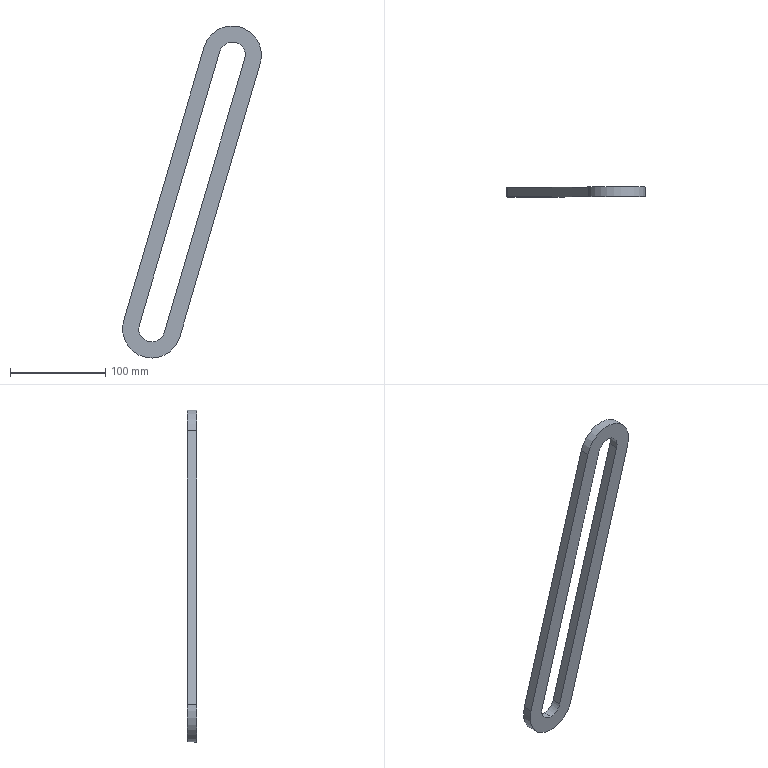Component | SolidWorks | Part3^CentrifugalDehydrator-1 | 1 solid | 12 faces | box 145.98 x 10 x 349.05 mm | volume 125654 mm3 | cylinder 6 | plane 6 | commonest cylinder face diameters 27.399 x3 61.399 x3
STEP:
#1=CARTESIAN_POINT('',(-12.559,-19.736,-16.297));
#2=VERTEX_POINT('',#1);
#3=CARTESIAN_POINT('',(-13.069,-19.736,-16.684));
#4=VERTEX_POINT('',#3);
#5=CARTESIAN_POINT('',(-13.077,-19.736,-16.145));
#6=DIRECTION('',(0.,1.,0.));
#7=DIRECTION('',(-0.01357,0.,0.9999));
#8=AXIS2_PLACEMENT_3D('',#5,#6,#7);
#9=CIRCLE('',#8,0.5393);
#10=EDGE_CURVE('',#2,#4,#9,.T.);
#11=ORIENTED_EDGE('',*,*,#10,.T.);
#12=CARTESIAN_POINT('',(-13.069,-20.13,-16.684));
#13=VERTEX_POINT('',#12);
#14=CARTESIAN_POINT('',(-13.069,-19.736,-16.684));
#15=DIRECTION('',(-0.,-1.,-0.));
#16=VECTOR('',#15,39.37);
#17=LINE('',#14,#16);
#18=EDGE_CURVE('',#4,#13,#17,.T.);
#19=ORIENTED_EDGE('',*,*,#18,.T.);
#20=CARTESIAN_POINT('',(-12.559,-20.13,-16.297));
#21=VERTEX_POINT('',#20);
#22=CARTESIAN_POINT('',(-13.077,-20.13,-16.145));
#23=DIRECTION('',(0.,1.,0.));
#24=DIRECTION('',(-0.01357,0.,0.9999));
#25=AXIS2_PLACEMENT_3D('',#22,#23,#24);
#26=CIRCLE('',#25,0.5393);
#27=EDGE_CURVE('',#21,#13,#26,.T.);
#28=ORIENTED_EDGE('',*,*,#27,.F.);
#29=CARTESIAN_POINT('',(-12.559,-19.736,-16.297));
#30=DIRECTION('',(-0.,-1.,-0.));
#31=VECTOR('',#30,39.37);
#32=LINE('',#29,#31);
#33=EDGE_CURVE('',#2,#21,#32,.T.);
#34=ORIENTED_EDGE('',*,*,#33,.F.);
#35=EDGE_LOOP('',(#11,#19,#28,#34));
#36=FACE_OUTER_BOUND('',#35,.T.);
#37=CARTESIAN_POINT('',(-13.077,-19.736,-16.145));
#38=DIRECTION('',(-0.,-1.,-0.));
#39=DIRECTION('',(0.01357,0.,-0.9999));
#40=AXIS2_PLACEMENT_3D('',#37,#38,#39);
#41=CYLINDRICAL_SURFACE('',#40,0.5393);
#42=ADVANCED_FACE('',(#36),#41,.F.);
#43=CARTESIAN_POINT('',(-13.06,-19.736,-17.353));
#44=VERTEX_POINT('',#43);
#45=CARTESIAN_POINT('',(-14.236,-19.736,-15.804));
#46=VERTEX_POINT('',#45);
#47=CARTESIAN_POINT('',(-13.077,-19.736,-16.145));
#48=DIRECTION('',(0.,1.,0.));
#49=DIRECTION('',(-0.01357,-0.,0.9999));
#50=AXIS2_PLACEMENT_3D('',#47,#48,#49);
#51=CIRCLE('',#50,1.209);
#52=EDGE_CURVE('',#44,#46,#51,.T.);
#53=ORIENTED_EDGE('',*,*,#52,.F.);
#54=CARTESIAN_POINT('',(-13.06,-20.13,-17.353));
#55=VERTEX_POINT('',#54);
#56=CARTESIAN_POINT('',(-13.06,-19.736,-17.353));
#57=DIRECTION('',(-0.,-1.,-0.));
#58=VECTOR('',#57,39.37);
#59=LINE('',#56,#58);
#60=EDGE_CURVE('',#44,#55,#59,.T.);
#61=ORIENTED_EDGE('',*,*,#60,.T.);
#62=CARTESIAN_POINT('',(-14.236,-20.13,-15.804));
#63=VERTEX_POINT('',#62);
#64=CARTESIAN_POINT('',(-13.077,-20.13,-16.145));
#65=DIRECTION('',(0.,1.,0.));
#66=DIRECTION('',(-0.01357,-0.,0.9999));
#67=AXIS2_PLACEMENT_3D('',#64,#65,#66);
#68=CIRCLE('',#67,1.209);
#69=EDGE_CURVE('',#55,#63,#68,.T.);
#70=ORIENTED_EDGE('',*,*,#69,.T.);
#71=CARTESIAN_POINT('',(-14.236,-19.736,-15.804));
#72=DIRECTION('',(-0.,-1.,-0.));
#73=VECTOR('',#72,39.37);
#74=LINE('',#71,#73);
#75=EDGE_CURVE('',#46,#63,#74,.T.);
#76=ORIENTED_EDGE('',*,*,#75,.F.);
#77=EDGE_LOOP('',(#53,#61,#70,#76));
#78=FACE_OUTER_BOUND('',#77,.T.);
#79=CARTESIAN_POINT('',(-13.077,-19.736,-16.145));
#80=DIRECTION('',(-0.,-1.,-0.));
#81=DIRECTION('',(0.01357,0.,-0.9999));
#82=AXIS2_PLACEMENT_3D('',#79,#80,#81);
#83=CYLINDRICAL_SURFACE('',#82,1.209);
#84=ADVANCED_FACE('',(#78),#83,.T.);
#85=CARTESIAN_POINT('',(-11.917,-19.736,-16.486));
#86=VERTEX_POINT('',#85);
#87=CARTESIAN_POINT('',(-13.077,-19.736,-16.145));
#88=DIRECTION('',(0.,1.,0.));
#89=DIRECTION('',(-0.01357,-0.,0.9999));
#90=AXIS2_PLACEMENT_3D('',#87,#88,#89);
#91=CIRCLE('',#90,1.209);
#92=EDGE_CURVE('',#86,#44,#91,.T.);
#93=ORIENTED_EDGE('',*,*,#92,.T.);
#94=ORIENTED_EDGE('',*,*,#52,.T.);
#95=CARTESIAN_POINT('',(-10.906,-19.736,-4.479));
#96=VERTEX_POINT('',#95);
#97=CARTESIAN_POINT('',(-14.236,-19.736,-15.804));
#98=DIRECTION('',(0.2821,-0.,0.9594));
#99=VECTOR('',#98,39.37);
#100=LINE('',#97,#99);
#101=EDGE_CURVE('',#46,#96,#100,.T.);
#102=ORIENTED_EDGE('',*,*,#101,.T.);
#103=CARTESIAN_POINT('',(-8.587,-19.736,-5.161));
#104=VERTEX_POINT('',#103);
#105=CARTESIAN_POINT('',(-9.747,-19.736,-4.82));
#106=DIRECTION('',(0.,1.,0.));
#107=DIRECTION('',(-0.01357,-0.,0.9999));
#108=AXIS2_PLACEMENT_3D('',#105,#106,#107);
#109=CIRCLE('',#108,1.209);
#110=EDGE_CURVE('',#96,#104,#109,.T.);
#111=ORIENTED_EDGE('',*,*,#110,.T.);
#112=CARTESIAN_POINT('',(-11.917,-19.736,-16.486));
#113=DIRECTION('',(-0.2821,0.,-0.9594));
#114=VECTOR('',#113,39.37);
#115=LINE('',#112,#114);
#116=EDGE_CURVE('',#104,#86,#115,.T.);
#117=ORIENTED_EDGE('',*,*,#116,.T.);
#118=EDGE_LOOP('',(#93,#94,#102,#111,#117));
#119=FACE_OUTER_BOUND('',#118,.T.);
#120=CARTESIAN_POINT('',(-13.594,-19.736,-15.992));
#121=VERTEX_POINT('',#120);
#122=CARTESIAN_POINT('',(-10.264,-19.736,-4.668));
#123=VERTEX_POINT('',#122);
#124=CARTESIAN_POINT('',(-13.594,-19.736,-15.992));
#125=DIRECTION('',(0.2821,-0.,0.9594));
#126=VECTOR('',#125,39.37);
#127=LINE('',#124,#126);
#128=EDGE_CURVE('',#121,#123,#127,.T.);
#129=ORIENTED_EDGE('',*,*,#128,.F.);
#130=CARTESIAN_POINT('',(-13.077,-19.736,-16.145));
#131=DIRECTION('',(0.,1.,0.));
#132=DIRECTION('',(-0.01357,0.,0.9999));
#133=AXIS2_PLACEMENT_3D('',#130,#131,#132);
#134=CIRCLE('',#133,0.5393);
#135=EDGE_CURVE('',#4,#121,#134,.T.);
#136=ORIENTED_EDGE('',*,*,#135,.F.);
#137=ORIENTED_EDGE('',*,*,#10,.F.);
#138=CARTESIAN_POINT('',(-9.229,-19.736,-4.972));
#139=VERTEX_POINT('',#138);
#140=CARTESIAN_POINT('',(-12.559,-19.736,-16.297));
#141=DIRECTION('',(-0.2821,0.,-0.9594));
#142=VECTOR('',#141,39.37);
#143=LINE('',#140,#142);
#144=EDGE_CURVE('',#139,#2,#143,.T.);
#145=ORIENTED_EDGE('',*,*,#144,.F.);
#146=CARTESIAN_POINT('',(-9.747,-19.736,-4.82));
#147=DIRECTION('',(0.,1.,0.));
#148=DIRECTION('',(-0.01357,0.,0.9999));
#149=AXIS2_PLACEMENT_3D('',#146,#147,#148);
#150=CIRCLE('',#149,0.5393);
#151=EDGE_CURVE('',#123,#139,#150,.T.);
#152=ORIENTED_EDGE('',*,*,#151,.F.);
#153=EDGE_LOOP('',(#129,#136,#137,#145,#152));
#154=FACE_BOUND('',#153,.T.);
#155=CARTESIAN_POINT('',(-13.077,-19.736,-16.145));
#156=DIRECTION('',(0.,1.,0.));
#157=DIRECTION('',(-0.01357,-0.,0.9999));
#158=AXIS2_PLACEMENT_3D('',#155,#156,#157);
#159=PLANE('',#158);
#160=ADVANCED_FACE('',(#119,#154),#159,.T.);
#161=CARTESIAN_POINT('',(-11.917,-20.13,-16.486));
#162=VERTEX_POINT('',#161);
#163=CARTESIAN_POINT('',(-13.077,-20.13,-16.145));
#164=DIRECTION('',(0.,1.,0.));
#165=DIRECTION('',(-0.01357,-0.,0.9999));
#166=AXIS2_PLACEMENT_3D('',#163,#164,#165);
#167=CIRCLE('',#166,1.209);
#168=EDGE_CURVE('',#162,#55,#167,.T.);
#169=ORIENTED_EDGE('',*,*,#168,.F.);
#170=CARTESIAN_POINT('',(-8.587,-20.13,-5.161));
#171=VERTEX_POINT('',#170);
#172=CARTESIAN_POINT('',(-11.917,-20.13,-16.486));
#173=DIRECTION('',(-0.2821,0.,-0.9594));
#174=VECTOR('',#173,39.37);
#175=LINE('',#172,#174);
#176=EDGE_CURVE('',#171,#162,#175,.T.);
#177=ORIENTED_EDGE('',*,*,#176,.F.);
#178=CARTESIAN_POINT('',(-10.906,-20.13,-4.479));
#179=VERTEX_POINT('',#178);
#180=CARTESIAN_POINT('',(-9.747,-20.13,-4.82));
#181=DIRECTION('',(0.,1.,0.));
#182=DIRECTION('',(-0.01357,-0.,0.9999));
#183=AXIS2_PLACEMENT_3D('',#180,#181,#182);
#184=CIRCLE('',#183,1.209);
#185=EDGE_CURVE('',#179,#171,#184,.T.);
#186=ORIENTED_EDGE('',*,*,#185,.F.);
#187=CARTESIAN_POINT('',(-14.236,-20.13,-15.804));
#188=DIRECTION('',(0.2821,-0.,0.9594));
#189=VECTOR('',#188,39.37);
#190=LINE('',#187,#189);
#191=EDGE_CURVE('',#63,#179,#190,.T.);
#192=ORIENTED_EDGE('',*,*,#191,.F.);
#193=ORIENTED_EDGE('',*,*,#69,.F.);
#194=EDGE_LOOP('',(#169,#177,#186,#192,#193));
#195=FACE_OUTER_BOUND('',#194,.T.);
#196=ORIENTED_EDGE('',*,*,#27,.T.);
#197=CARTESIAN_POINT('',(-13.594,-20.13,-15.992));
#198=VERTEX_POINT('',#197);
#199=CARTESIAN_POINT('',(-13.077,-20.13,-16.145));
#200=DIRECTION('',(0.,1.,0.));
#201=DIRECTION('',(-0.01357,0.,0.9999));
#202=AXIS2_PLACEMENT_3D('',#199,#200,#201);
#203=CIRCLE('',#202,0.5393);
#204=EDGE_CURVE('',#13,#198,#203,.T.);
#205=ORIENTED_EDGE('',*,*,#204,.T.);
#206=CARTESIAN_POINT('',(-10.264,-20.13,-4.668));
#207=VERTEX_POINT('',#206);
#208=CARTESIAN_POINT('',(-13.594,-20.13,-15.992));
#209=DIRECTION('',(0.2821,-0.,0.9594));
#210=VECTOR('',#209,39.37);
#211=LINE('',#208,#210);
#212=EDGE_CURVE('',#198,#207,#211,.T.);
#213=ORIENTED_EDGE('',*,*,#212,.T.);
#214=CARTESIAN_POINT('',(-9.229,-20.13,-4.972));
#215=VERTEX_POINT('',#214);
#216=CARTESIAN_POINT('',(-9.747,-20.13,-4.82));
#217=DIRECTION('',(0.,1.,0.));
#218=DIRECTION('',(-0.01357,0.,0.9999));
#219=AXIS2_PLACEMENT_3D('',#216,#217,#218);
#220=CIRCLE('',#219,0.5393);
#221=EDGE_CURVE('',#207,#215,#220,.T.);
#222=ORIENTED_EDGE('',*,*,#221,.T.);
#223=CARTESIAN_POINT('',(-12.559,-20.13,-16.297));
#224=DIRECTION('',(-0.2821,0.,-0.9594));
#225=VECTOR('',#224,39.37);
#226=LINE('',#223,#225);
#227=EDGE_CURVE('',#215,#21,#226,.T.);
#228=ORIENTED_EDGE('',*,*,#227,.T.);
#229=EDGE_LOOP('',(#196,#205,#213,#222,#228));
#230=FACE_BOUND('',#229,.T.);
#231=CARTESIAN_POINT('',(-13.077,-20.13,-16.145));
#232=DIRECTION('',(0.,1.,0.));
#233=DIRECTION('',(-0.01357,-0.,0.9999));
#234=AXIS2_PLACEMENT_3D('',#231,#232,#233);
#235=PLANE('',#234);
#236=ADVANCED_FACE('',(#195,#230),#235,.F.);
#237=ORIENTED_EDGE('',*,*,#60,.F.);
#238=ORIENTED_EDGE('',*,*,#92,.F.);
#239=CARTESIAN_POINT('',(-11.917,-19.736,-16.486));
#240=DIRECTION('',(-0.,-1.,-0.));
#241=VECTOR('',#240,39.37);
#242=LINE('',#239,#241);
#243=EDGE_CURVE('',#86,#162,#242,.T.);
#244=ORIENTED_EDGE('',*,*,#243,.T.);
#245=ORIENTED_EDGE('',*,*,#168,.T.);
#246=EDGE_LOOP('',(#237,#238,#244,#245));
#247=FACE_OUTER_BOUND('',#246,.T.);
#248=CARTESIAN_POINT('',(-13.077,-19.736,-16.145));
#249=DIRECTION('',(-0.,-1.,-0.));
#250=DIRECTION('',(0.01357,0.,-0.9999));
#251=AXIS2_PLACEMENT_3D('',#248,#249,#250);
#252=CYLINDRICAL_SURFACE('',#251,1.209);
#253=ADVANCED_FACE('',(#247),#252,.T.);
#254=ORIENTED_EDGE('',*,*,#191,.T.);
#255=CARTESIAN_POINT('',(-10.906,-19.736,-4.479));
#256=DIRECTION('',(-0.,-1.,-0.));
#257=VECTOR('',#256,39.37);
#258=LINE('',#255,#257);
#259=EDGE_CURVE('',#96,#179,#258,.T.);
#260=ORIENTED_EDGE('',*,*,#259,.F.);
#261=ORIENTED_EDGE('',*,*,#101,.F.);
#262=ORIENTED_EDGE('',*,*,#75,.T.);
#263=EDGE_LOOP('',(#254,#260,#261,#262));
#264=FACE_OUTER_BOUND('',#263,.T.);
#265=CARTESIAN_POINT('',(-14.236,-19.736,-15.804));
#266=DIRECTION('',(0.9594,0.,-0.2821));
#267=DIRECTION('',(-0.2821,0.,-0.9594));
#268=AXIS2_PLACEMENT_3D('',#265,#266,#267);
#269=PLANE('',#268);
#270=ADVANCED_FACE('',(#264),#269,.F.);
#271=ORIENTED_EDGE('',*,*,#185,.T.);
#272=CARTESIAN_POINT('',(-8.587,-19.736,-5.161));
#273=DIRECTION('',(-0.,-1.,-0.));
#274=VECTOR('',#273,39.37);
#275=LINE('',#272,#274);
#276=EDGE_CURVE('',#104,#171,#275,.T.);
#277=ORIENTED_EDGE('',*,*,#276,.F.);
#278=ORIENTED_EDGE('',*,*,#110,.F.);
#279=ORIENTED_EDGE('',*,*,#259,.T.);
#280=EDGE_LOOP('',(#271,#277,#278,#279));
#281=FACE_OUTER_BOUND('',#280,.T.);
#282=CARTESIAN_POINT('',(-9.747,-19.736,-4.82));
#283=DIRECTION('',(-0.,-1.,-0.));
#284=DIRECTION('',(0.01357,0.,-0.9999));
#285=AXIS2_PLACEMENT_3D('',#282,#283,#284);
#286=CYLINDRICAL_SURFACE('',#285,1.209);
#287=ADVANCED_FACE('',(#281),#286,.T.);
#288=ORIENTED_EDGE('',*,*,#176,.T.);
#289=ORIENTED_EDGE('',*,*,#243,.F.);
#290=ORIENTED_EDGE('',*,*,#116,.F.);
#291=ORIENTED_EDGE('',*,*,#276,.T.);
#292=EDGE_LOOP('',(#288,#289,#290,#291));
#293=FACE_OUTER_BOUND('',#292,.T.);
#294=CARTESIAN_POINT('',(-11.917,-19.736,-16.486));
#295=DIRECTION('',(-0.9594,-0.,0.2821));
#296=DIRECTION('',(0.2821,-0.,0.9594));
#297=AXIS2_PLACEMENT_3D('',#294,#295,#296);
#298=PLANE('',#297);
#299=ADVANCED_FACE('',(#293),#298,.F.);
#300=ORIENTED_EDGE('',*,*,#18,.F.);
#301=ORIENTED_EDGE('',*,*,#135,.T.);
#302=CARTESIAN_POINT('',(-13.594,-19.736,-15.992));
#303=DIRECTION('',(-0.,-1.,-0.));
#304=VECTOR('',#303,39.37);
#305=LINE('',#302,#304);
#306=EDGE_CURVE('',#121,#198,#305,.T.);
#307=ORIENTED_EDGE('',*,*,#306,.T.);
#308=ORIENTED_EDGE('',*,*,#204,.F.);
#309=EDGE_LOOP('',(#300,#301,#307,#308));
#310=FACE_OUTER_BOUND('',#309,.T.);
#311=CARTESIAN_POINT('',(-13.077,-19.736,-16.145));
#312=DIRECTION('',(-0.,-1.,-0.));
#313=DIRECTION('',(0.01357,0.,-0.9999));
#314=AXIS2_PLACEMENT_3D('',#311,#312,#313);
#315=CYLINDRICAL_SURFACE('',#314,0.5393);
#316=ADVANCED_FACE('',(#310),#315,.F.);
#317=ORIENTED_EDGE('',*,*,#212,.F.);
#318=ORIENTED_EDGE('',*,*,#306,.F.);
#319=ORIENTED_EDGE('',*,*,#128,.T.);
#320=CARTESIAN_POINT('',(-10.264,-19.736,-4.668));
#321=DIRECTION('',(-0.,-1.,-0.));
#322=VECTOR('',#321,39.37);
#323=LINE('',#320,#322);
#324=EDGE_CURVE('',#123,#207,#323,.T.);
#325=ORIENTED_EDGE('',*,*,#324,.T.);
#326=EDGE_LOOP('',(#317,#318,#319,#325));
#327=FACE_OUTER_BOUND('',#326,.T.);
#328=CARTESIAN_POINT('',(-13.594,-19.736,-15.992));
#329=DIRECTION('',(0.9594,0.,-0.2821));
#330=DIRECTION('',(-0.2821,0.,-0.9594));
#331=AXIS2_PLACEMENT_3D('',#328,#329,#330);
#332=PLANE('',#331);
#333=ADVANCED_FACE('',(#327),#332,.T.);
#334=ORIENTED_EDGE('',*,*,#221,.F.);
#335=ORIENTED_EDGE('',*,*,#324,.F.);
#336=ORIENTED_EDGE('',*,*,#151,.T.);
#337=CARTESIAN_POINT('',(-9.229,-19.736,-4.972));
#338=DIRECTION('',(-0.,-1.,-0.));
#339=VECTOR('',#338,39.37);
#340=LINE('',#337,#339);
#341=EDGE_CURVE('',#139,#215,#340,.T.);
#342=ORIENTED_EDGE('',*,*,#341,.T.);
#343=EDGE_LOOP('',(#334,#335,#336,#342));
#344=FACE_OUTER_BOUND('',#343,.T.);
#345=CARTESIAN_POINT('',(-9.747,-19.736,-4.82));
#346=DIRECTION('',(-0.,-1.,-0.));
#347=DIRECTION('',(0.01357,0.,-0.9999));
#348=AXIS2_PLACEMENT_3D('',#345,#346,#347);
#349=CYLINDRICAL_SURFACE('',#348,0.5393);
#350=ADVANCED_FACE('',(#344),#349,.F.);
#351=ORIENTED_EDGE('',*,*,#227,.F.);
#352=ORIENTED_EDGE('',*,*,#341,.F.);
#353=ORIENTED_EDGE('',*,*,#144,.T.);
#354=ORIENTED_EDGE('',*,*,#33,.T.);
#355=EDGE_LOOP('',(#351,#352,#353,#354));
#356=FACE_OUTER_BOUND('',#355,.T.);
#357=CARTESIAN_POINT('',(-12.559,-19.736,-16.297));
#358=DIRECTION('',(-0.9594,-0.,0.2821));
#359=DIRECTION('',(0.2821,-0.,0.9594));
#360=AXIS2_PLACEMENT_3D('',#357,#358,#359);
#361=PLANE('',#360);
#362=ADVANCED_FACE('',(#356),#361,.T.);
#363=CLOSED_SHELL('',(#42,#84,#160,#236,#253,#270,#287,#299,#316,#333,#350,#362));
#364=MANIFOLD_SOLID_BREP('',#363);
#365=CARTESIAN_POINT('',(0.,0.,0.));
#366=DIRECTION('',(0.,0.,1.));
#367=DIRECTION('',(1.,0.,0.));
#368=AXIS2_PLACEMENT_3D('',#365,#366,#367);
#369=(LENGTH_UNIT()NAMED_UNIT(*)SI_UNIT($,.METRE.));
#370=LENGTH_MEASURE_WITH_UNIT(LENGTH_MEASURE(0.0254),#369);
#371=DIMENSIONAL_EXPONENTS(1.,0.,0.,0.,0.,0.,0.);
#372=(CONVERSION_BASED_UNIT('',#370)LENGTH_UNIT()NAMED_UNIT(#371));
#373=UNCERTAINTY_MEASURE_WITH_UNIT(LENGTH_MEASURE(0.00001),#372,'','');
#374=(NAMED_UNIT(*)PLANE_ANGLE_UNIT()SI_UNIT($,.RADIAN.));
#375=(NAMED_UNIT(*)SI_UNIT($,.STERADIAN.)SOLID_ANGLE_UNIT());
#376=(GEOMETRIC_REPRESENTATION_CONTEXT(3)GLOBAL_UNCERTAINTY_ASSIGNED_CONTEXT((#373))GLOBAL_UNIT_ASSIGNED_CONTEXT((#372,#374,#375))REPRESENTATION_CONTEXT('',''));
#377=ADVANCED_BREP_SHAPE_REPRESENTATION('',(#364,#368),#376);
#378=COLOUR_RGB('',0.7922,0.8196,0.9333);
#379=FILL_AREA_STYLE_COLOUR('',#378);
#380=FILL_AREA_STYLE('',(#379));
#381=SURFACE_STYLE_FILL_AREA(#380);
#382=SURFACE_SIDE_STYLE('',(#381));
#383=SURFACE_STYLE_USAGE(.BOTH.,#382);
#384=PRESENTATION_STYLE_ASSIGNMENT((#383));
#385=STYLED_ITEM('',(#384),#364);
#386=(LENGTH_UNIT()NAMED_UNIT(*)SI_UNIT($,.METRE.));
#387=LENGTH_MEASURE_WITH_UNIT(LENGTH_MEASURE(0.0254),#386);
#388=DIMENSIONAL_EXPONENTS(1.,0.,0.,0.,0.,0.,0.);
#389=(CONVERSION_BASED_UNIT('',#387)LENGTH_UNIT()NAMED_UNIT(#388));
#390=UNCERTAINTY_MEASURE_WITH_UNIT(LENGTH_MEASURE(0.00001),#389,'','');
#391=(NAMED_UNIT(*)PLANE_ANGLE_UNIT()SI_UNIT($,.RADIAN.));
#392=(NAMED_UNIT(*)SI_UNIT($,.STERADIAN.)SOLID_ANGLE_UNIT());
#393=(GEOMETRIC_REPRESENTATION_CONTEXT(3)GLOBAL_UNCERTAINTY_ASSIGNED_CONTEXT((#390))GLOBAL_UNIT_ASSIGNED_CONTEXT((#389,#391,#392))REPRESENTATION_CONTEXT('',''));
#394=MECHANICAL_DESIGN_GEOMETRIC_PRESENTATION_REPRESENTATION('',(#385),#393);
#395=PRESENTATION_LAYER_ASSIGNMENT('','',(#385));